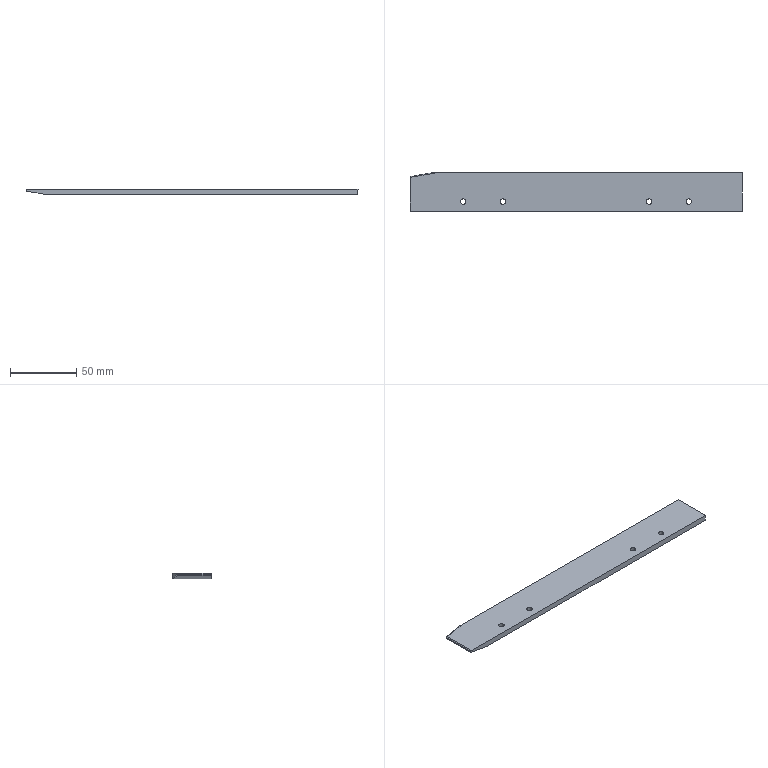Component | SolidWorks | 2SZT-0-009-3 | 1 solid | 26 faces | box 250 x 29 x 4.51 mm | volume 31578 mm3 | cylinder 15 | plane 8 | sphere 2 | spline 1 | commonest cylinder face diameters 1 x6 4.01 x4 4.2 x4 20 x1
STEP:
#1=COLOUR_RGB('',0.7922,0.8196,0.9333);
#2=FILL_AREA_STYLE_COLOUR('',#1);
#3=FILL_AREA_STYLE('',(#2));
#4=SURFACE_STYLE_FILL_AREA(#3);
#5=SURFACE_SIDE_STYLE('',(#4));
#6=SURFACE_STYLE_USAGE(.BOTH.,#5);
#7=PRESENTATION_STYLE_ASSIGNMENT((#6));
#8=CARTESIAN_POINT('',(34.695,16.445,-10.866));
#9=VERTEX_POINT('',#8);
#10=CARTESIAN_POINT('',(34.853,16.445,-10.866));
#11=VERTEX_POINT('',#10);
#12=CARTESIAN_POINT('',(34.774,16.445,-10.866));
#13=DIRECTION('',(0.00002551,0.,1.));
#14=DIRECTION('',(1.,0.,-0.00002551));
#15=AXIS2_PLACEMENT_3D('',#12,#13,#14);
#16=CIRCLE('',#15,0.07894);
#17=EDGE_CURVE('',#9,#11,#16,.T.);
#18=ORIENTED_EDGE('',*,*,#17,.F.);
#19=CARTESIAN_POINT('',(34.695,16.445,-10.689));
#20=VERTEX_POINT('',#19);
#21=CARTESIAN_POINT('',(34.695,16.445,-10.689));
#22=DIRECTION('',(0.00002551,0.,1.));
#23=VECTOR('',#22,39.37);
#24=LINE('',#21,#23);
#25=EDGE_CURVE('',#9,#20,#24,.T.);
#26=ORIENTED_EDGE('',*,*,#25,.T.);
#27=CARTESIAN_POINT('',(34.853,16.445,-10.689));
#28=VERTEX_POINT('',#27);
#29=CARTESIAN_POINT('',(34.774,16.445,-10.689));
#30=DIRECTION('',(0.00002551,0.,1.));
#31=DIRECTION('',(1.,0.,-0.00002551));
#32=AXIS2_PLACEMENT_3D('',#29,#30,#31);
#33=CIRCLE('',#32,0.07894);
#34=EDGE_CURVE('',#20,#28,#33,.T.);
#35=ORIENTED_EDGE('',*,*,#34,.T.);
#36=CARTESIAN_POINT('',(34.853,16.445,-10.689));
#37=DIRECTION('',(0.00002551,0.,1.));
#38=VECTOR('',#37,39.37);
#39=LINE('',#36,#38);
#40=EDGE_CURVE('',#11,#28,#39,.T.);
#41=ORIENTED_EDGE('',*,*,#40,.F.);
#42=EDGE_LOOP('',(#18,#26,#35,#41));
#43=FACE_OUTER_BOUND('',#42,.T.);
#44=CARTESIAN_POINT('',(34.774,16.445,-10.689));
#45=DIRECTION('',(0.00002551,0.,1.));
#46=DIRECTION('',(1.,0.,-0.00002551));
#47=AXIS2_PLACEMENT_3D('',#44,#45,#46);
#48=CYLINDRICAL_SURFACE('',#47,0.07894);
#49=ADVANCED_FACE('',(#43),#48,.F.);
#50=CARTESIAN_POINT('',(41.388,16.445,-10.866));
#51=VERTEX_POINT('',#50);
#52=CARTESIAN_POINT('',(41.546,16.445,-10.866));
#53=VERTEX_POINT('',#52);
#54=CARTESIAN_POINT('',(41.467,16.445,-10.866));
#55=DIRECTION('',(0.00002551,0.,1.));
#56=DIRECTION('',(1.,0.,-0.00002551));
#57=AXIS2_PLACEMENT_3D('',#54,#55,#56);
#58=CIRCLE('',#57,0.07894);
#59=EDGE_CURVE('',#51,#53,#58,.T.);
#60=ORIENTED_EDGE('',*,*,#59,.F.);
#61=CARTESIAN_POINT('',(41.388,16.445,-10.689));
#62=VERTEX_POINT('',#61);
#63=CARTESIAN_POINT('',(41.388,16.445,-10.689));
#64=DIRECTION('',(0.00002551,0.,1.));
#65=VECTOR('',#64,39.37);
#66=LINE('',#63,#65);
#67=EDGE_CURVE('',#51,#62,#66,.T.);
#68=ORIENTED_EDGE('',*,*,#67,.T.);
#69=CARTESIAN_POINT('',(41.546,16.445,-10.689));
#70=VERTEX_POINT('',#69);
#71=CARTESIAN_POINT('',(41.467,16.445,-10.689));
#72=DIRECTION('',(0.00002551,0.,1.));
#73=DIRECTION('',(1.,0.,-0.00002551));
#74=AXIS2_PLACEMENT_3D('',#71,#72,#73);
#75=CIRCLE('',#74,0.07894);
#76=EDGE_CURVE('',#62,#70,#75,.T.);
#77=ORIENTED_EDGE('',*,*,#76,.T.);
#78=CARTESIAN_POINT('',(41.546,16.445,-10.689));
#79=DIRECTION('',(0.00002551,0.,1.));
#80=VECTOR('',#79,39.37);
#81=LINE('',#78,#80);
#82=EDGE_CURVE('',#53,#70,#81,.T.);
#83=ORIENTED_EDGE('',*,*,#82,.F.);
#84=EDGE_LOOP('',(#60,#68,#77,#83));
#85=FACE_OUTER_BOUND('',#84,.T.);
#86=CARTESIAN_POINT('',(41.467,16.445,-10.689));
#87=DIRECTION('',(0.00002551,0.,1.));
#88=DIRECTION('',(1.,0.,-0.00002551));
#89=AXIS2_PLACEMENT_3D('',#86,#87,#88);
#90=CYLINDRICAL_SURFACE('',#89,0.07894);
#91=ADVANCED_FACE('',(#85),#90,.F.);
#92=CARTESIAN_POINT('',(35.873,16.445,-10.689));
#93=VERTEX_POINT('',#92);
#94=CARTESIAN_POINT('',(36.038,16.445,-10.689));
#95=VERTEX_POINT('',#94);
#96=CARTESIAN_POINT('',(35.955,16.445,-10.689));
#97=DIRECTION('',(0.00002551,0.,1.));
#98=DIRECTION('',(1.,0.,-0.00002551));
#99=AXIS2_PLACEMENT_3D('',#96,#97,#98);
#100=CIRCLE('',#99,0.08268);
#101=EDGE_CURVE('',#93,#95,#100,.T.);
#102=ORIENTED_EDGE('',*,*,#101,.T.);
#103=CARTESIAN_POINT('',(36.038,16.445,-10.866));
#104=VERTEX_POINT('',#103);
#105=CARTESIAN_POINT('',(36.038,16.445,-10.866));
#106=DIRECTION('',(-0.00002551,-0.,-1.));
#107=VECTOR('',#106,39.37);
#108=LINE('',#105,#107);
#109=EDGE_CURVE('',#95,#104,#108,.T.);
#110=ORIENTED_EDGE('',*,*,#109,.T.);
#111=CARTESIAN_POINT('',(35.873,16.445,-10.866));
#112=VERTEX_POINT('',#111);
#113=CARTESIAN_POINT('',(35.955,16.445,-10.866));
#114=DIRECTION('',(-0.00002551,-0.,-1.));
#115=DIRECTION('',(-1.,0.,0.00002551));
#116=AXIS2_PLACEMENT_3D('',#113,#114,#115);
#117=CIRCLE('',#116,0.08268);
#118=EDGE_CURVE('',#104,#112,#117,.T.);
#119=ORIENTED_EDGE('',*,*,#118,.T.);
#120=CARTESIAN_POINT('',(35.873,16.445,-10.866));
#121=DIRECTION('',(-0.00002551,-0.,-1.));
#122=VECTOR('',#121,39.37);
#123=LINE('',#120,#122);
#124=EDGE_CURVE('',#93,#112,#123,.T.);
#125=ORIENTED_EDGE('',*,*,#124,.F.);
#126=EDGE_LOOP('',(#102,#110,#119,#125));
#127=FACE_OUTER_BOUND('',#126,.T.);
#128=CARTESIAN_POINT('',(35.955,16.445,-10.866));
#129=DIRECTION('',(-0.00002551,-0.,-1.));
#130=DIRECTION('',(-1.,0.,0.00002551));
#131=AXIS2_PLACEMENT_3D('',#128,#129,#130);
#132=CYLINDRICAL_SURFACE('',#131,0.08268);
#133=ADVANCED_FACE('',(#127),#132,.F.);
#134=CARTESIAN_POINT('',(40.203,16.445,-10.689));
#135=VERTEX_POINT('',#134);
#136=CARTESIAN_POINT('',(40.369,16.445,-10.689));
#137=VERTEX_POINT('',#136);
#138=CARTESIAN_POINT('',(40.286,16.445,-10.689));
#139=DIRECTION('',(0.00002551,0.,1.));
#140=DIRECTION('',(1.,0.,-0.00002551));
#141=AXIS2_PLACEMENT_3D('',#138,#139,#140);
#142=CIRCLE('',#141,0.08268);
#143=EDGE_CURVE('',#135,#137,#142,.T.);
#144=ORIENTED_EDGE('',*,*,#143,.T.);
#145=CARTESIAN_POINT('',(40.369,16.445,-10.866));
#146=VERTEX_POINT('',#145);
#147=CARTESIAN_POINT('',(40.369,16.445,-10.866));
#148=DIRECTION('',(-0.00002551,-0.,-1.));
#149=VECTOR('',#148,39.37);
#150=LINE('',#147,#149);
#151=EDGE_CURVE('',#137,#146,#150,.T.);
#152=ORIENTED_EDGE('',*,*,#151,.T.);
#153=CARTESIAN_POINT('',(40.203,16.445,-10.866));
#154=VERTEX_POINT('',#153);
#155=CARTESIAN_POINT('',(40.286,16.445,-10.866));
#156=DIRECTION('',(-0.00002551,-0.,-1.));
#157=DIRECTION('',(-1.,0.,0.00002551));
#158=AXIS2_PLACEMENT_3D('',#155,#156,#157);
#159=CIRCLE('',#158,0.08268);
#160=EDGE_CURVE('',#146,#154,#159,.T.);
#161=ORIENTED_EDGE('',*,*,#160,.T.);
#162=CARTESIAN_POINT('',(40.203,16.445,-10.866));
#163=DIRECTION('',(-0.00002551,-0.,-1.));
#164=VECTOR('',#163,39.37);
#165=LINE('',#162,#164);
#166=EDGE_CURVE('',#135,#154,#165,.T.);
#167=ORIENTED_EDGE('',*,*,#166,.F.);
#168=EDGE_LOOP('',(#144,#152,#161,#167));
#169=FACE_OUTER_BOUND('',#168,.T.);
#170=CARTESIAN_POINT('',(40.286,16.445,-10.866));
#171=DIRECTION('',(-0.00002551,-0.,-1.));
#172=DIRECTION('',(-1.,0.,0.00002551));
#173=AXIS2_PLACEMENT_3D('',#170,#171,#172);
#174=CYLINDRICAL_SURFACE('',#173,0.08268);
#175=ADVANCED_FACE('',(#169),#174,.F.);
#176=CARTESIAN_POINT('',(43.042,17.302,-10.689));
#177=VERTEX_POINT('',#176);
#178=CARTESIAN_POINT('',(43.042,16.16,-10.689));
#179=VERTEX_POINT('',#178);
#180=CARTESIAN_POINT('',(43.042,16.16,-10.689));
#181=DIRECTION('',(-0.,-1.,0.));
#182=VECTOR('',#181,39.37);
#183=LINE('',#180,#182);
#184=EDGE_CURVE('',#177,#179,#183,.T.);
#185=ORIENTED_EDGE('',*,*,#184,.T.);
#186=CARTESIAN_POINT('',(43.042,16.16,-10.866));
#187=VERTEX_POINT('',#186);
#188=CARTESIAN_POINT('',(43.042,16.16,-10.866));
#189=DIRECTION('',(0.00002551,0.,1.));
#190=VECTOR('',#189,39.37);
#191=LINE('',#188,#190);
#192=EDGE_CURVE('',#187,#179,#191,.T.);
#193=ORIENTED_EDGE('',*,*,#192,.F.);
#194=CARTESIAN_POINT('',(43.042,17.302,-10.866));
#195=VERTEX_POINT('',#194);
#196=CARTESIAN_POINT('',(43.042,16.16,-10.866));
#197=DIRECTION('',(-0.,-1.,0.));
#198=VECTOR('',#197,39.37);
#199=LINE('',#196,#198);
#200=EDGE_CURVE('',#195,#187,#199,.T.);
#201=ORIENTED_EDGE('',*,*,#200,.F.);
#202=CARTESIAN_POINT('',(43.042,17.302,-10.866));
#203=DIRECTION('',(0.00002551,0.,1.));
#204=VECTOR('',#203,39.37);
#205=LINE('',#202,#204);
#206=EDGE_CURVE('',#195,#177,#205,.T.);
#207=ORIENTED_EDGE('',*,*,#206,.T.);
#208=EDGE_LOOP('',(#185,#193,#201,#207));
#209=FACE_OUTER_BOUND('',#208,.T.);
#210=CARTESIAN_POINT('',(43.042,16.16,-10.866));
#211=DIRECTION('',(-1.,0.,0.00002551));
#212=DIRECTION('',(0.00002551,0.,1.));
#213=AXIS2_PLACEMENT_3D('',#210,#211,#212);
#214=PLANE('',#213);
#215=ADVANCED_FACE('',(#209),#214,.F.);
#216=CARTESIAN_POINT('',(33.219,16.16,-10.689));
#217=VERTEX_POINT('',#216);
#218=CARTESIAN_POINT('',(43.042,16.16,-10.689));
#219=DIRECTION('',(-1.,0.,0.00002551));
#220=VECTOR('',#219,39.37);
#221=LINE('',#218,#220);
#222=EDGE_CURVE('',#179,#217,#221,.T.);
#223=ORIENTED_EDGE('',*,*,#222,.T.);
#224=CARTESIAN_POINT('',(33.199,16.16,-10.708));
#225=VERTEX_POINT('',#224);
#226=CARTESIAN_POINT('',(33.219,16.16,-10.708));
#227=DIRECTION('',(-0.,-1.,0.));
#228=DIRECTION('',(-0.00002551,0.,-1.));
#229=AXIS2_PLACEMENT_3D('',#226,#227,#228);
#230=CIRCLE('',#229,0.01969);
#231=EDGE_CURVE('',#217,#225,#230,.T.);
#232=ORIENTED_EDGE('',*,*,#231,.T.);
#233=CARTESIAN_POINT('',(33.199,16.16,-10.731));
#234=VERTEX_POINT('',#233);
#235=CARTESIAN_POINT('',(33.199,16.16,-10.866));
#236=DIRECTION('',(0.00002551,0.,1.));
#237=VECTOR('',#236,39.37);
#238=LINE('',#235,#237);
#239=EDGE_CURVE('',#234,#225,#238,.T.);
#240=ORIENTED_EDGE('',*,*,#239,.F.);
#241=CARTESIAN_POINT('',(33.216,16.16,-10.751));
#242=VERTEX_POINT('',#241);
#243=CARTESIAN_POINT('',(33.219,16.16,-10.731));
#244=DIRECTION('',(-0.,-1.,0.));
#245=DIRECTION('',(-0.00002551,0.,-1.));
#246=AXIS2_PLACEMENT_3D('',#243,#244,#245);
#247=CIRCLE('',#246,0.01969);
#248=EDGE_CURVE('',#234,#242,#247,.T.);
#249=ORIENTED_EDGE('',*,*,#248,.T.);
#250=CARTESIAN_POINT('',(33.835,16.16,-10.86));
#251=VERTEX_POINT('',#250);
#252=CARTESIAN_POINT('',(33.869,16.16,-10.866));
#253=DIRECTION('',(0.9848,-0.,-0.1737));
#254=VECTOR('',#253,39.37);
#255=LINE('',#252,#254);
#256=EDGE_CURVE('',#242,#251,#255,.T.);
#257=ORIENTED_EDGE('',*,*,#256,.T.);
#258=CARTESIAN_POINT('',(33.904,16.16,-10.866));
#259=VERTEX_POINT('',#258);
#260=CARTESIAN_POINT('',(33.904,16.16,-10.472));
#261=DIRECTION('',(-0.,-1.,0.));
#262=DIRECTION('',(-0.00002551,0.,-1.));
#263=AXIS2_PLACEMENT_3D('',#260,#261,#262);
#264=CIRCLE('',#263,0.3937);
#265=EDGE_CURVE('',#251,#259,#264,.T.);
#266=ORIENTED_EDGE('',*,*,#265,.T.);
#267=CARTESIAN_POINT('',(43.042,16.16,-10.866));
#268=DIRECTION('',(-1.,0.,0.00002551));
#269=VECTOR('',#268,39.37);
#270=LINE('',#267,#269);
#271=EDGE_CURVE('',#187,#259,#270,.T.);
#272=ORIENTED_EDGE('',*,*,#271,.F.);
#273=ORIENTED_EDGE('',*,*,#192,.T.);
#274=EDGE_LOOP('',(#223,#232,#240,#249,#257,#266,#272,#273));
#275=FACE_OUTER_BOUND('',#274,.T.);
#276=CARTESIAN_POINT('',(43.042,16.16,-10.866));
#277=DIRECTION('',(0.,1.,-0.));
#278=DIRECTION('',(-0.00002551,-0.,-1.));
#279=AXIS2_PLACEMENT_3D('',#276,#277,#278);
#280=PLANE('',#279);
#281=ADVANCED_FACE('',(#275),#280,.F.);
#282=CARTESIAN_POINT('',(33.199,17.167,-10.708));
#283=VERTEX_POINT('',#282);
#284=CARTESIAN_POINT('',(33.199,17.184,-10.708));
#285=DIRECTION('',(0.,1.,-0.));
#286=VECTOR('',#285,39.37);
#287=LINE('',#284,#286);
#288=EDGE_CURVE('',#225,#283,#287,.T.);
#289=ORIENTED_EDGE('',*,*,#288,.T.);
#290=CARTESIAN_POINT('',(33.199,17.167,-10.731));
#291=VERTEX_POINT('',#290);
#292=CARTESIAN_POINT('',(33.199,17.167,-10.731));
#293=DIRECTION('',(-0.00002551,-0.,-1.));
#294=VECTOR('',#293,39.37);
#295=LINE('',#292,#294);
#296=EDGE_CURVE('',#283,#291,#295,.T.);
#297=ORIENTED_EDGE('',*,*,#296,.T.);
#298=CARTESIAN_POINT('',(33.199,16.16,-10.731));
#299=DIRECTION('',(-0.,-1.,0.));
#300=VECTOR('',#299,39.37);
#301=LINE('',#298,#300);
#302=EDGE_CURVE('',#291,#234,#301,.T.);
#303=ORIENTED_EDGE('',*,*,#302,.T.);
#304=ORIENTED_EDGE('',*,*,#239,.T.);
#305=EDGE_LOOP('',(#289,#297,#303,#304));
#306=FACE_OUTER_BOUND('',#305,.T.);
#307=CARTESIAN_POINT('',(33.199,16.16,-10.866));
#308=DIRECTION('',(1.,-0.,-0.00002551));
#309=DIRECTION('',(-0.00002551,-0.,-1.));
#310=AXIS2_PLACEMENT_3D('',#307,#308,#309);
#311=PLANE('',#310);
#312=ADVANCED_FACE('',(#306),#311,.F.);
#313=CARTESIAN_POINT('',(33.983,17.302,-10.866));
#314=VERTEX_POINT('',#313);
#315=CARTESIAN_POINT('',(33.901,17.302,-10.86));
#316=VERTEX_POINT('',#315);
#317=CARTESIAN_POINT('',(33.983,17.302,-10.866));
#318=CARTESIAN_POINT('',(33.952,17.302,-10.866));
#319=CARTESIAN_POINT('',(33.923,17.302,-10.864));
#320=CARTESIAN_POINT('',(33.901,17.302,-10.86));
#321=(BOUNDED_CURVE()B_SPLINE_CURVE(3,(#317,#318,#319,#320),.UNSPECIFIED.,.F.,.T.)B_SPLINE_CURVE_WITH_KNOTS((4,4),(4.712,5.513),.UNSPECIFIED.)CURVE()GEOMETRIC_REPRESENTATION_ITEM()RATIONAL_B_SPLINE_CURVE((1.,0.9473,0.9473,1.))REPRESENTATION_ITEM(''));
#322=EDGE_CURVE('',#314,#316,#321,.T.);
#323=ORIENTED_EDGE('',*,*,#322,.T.);
#324=CARTESIAN_POINT('',(33.869,17.302,-10.845));
#325=VERTEX_POINT('',#324);
#326=CARTESIAN_POINT('',(33.901,17.302,-10.86));
#327=CARTESIAN_POINT('',(33.895,17.302,-10.859));
#328=CARTESIAN_POINT('',(33.889,17.302,-10.857));
#329=CARTESIAN_POINT('',(33.881,17.302,-10.854));
#330=CARTESIAN_POINT('',(33.878,17.302,-10.853));
#331=CARTESIAN_POINT('',(33.874,17.302,-10.851));
#332=CARTESIAN_POINT('',(33.873,17.302,-10.85));
#333=CARTESIAN_POINT('',(33.87,17.302,-10.848));
#334=CARTESIAN_POINT('',(33.869,17.302,-10.846));
#335=CARTESIAN_POINT('',(33.869,17.302,-10.845));
#336=B_SPLINE_CURVE_WITH_KNOTS('',3,(#326,#327,#328,#329,#330,#331,#332,#333,#334,#335),.UNSPECIFIED.,.F.,.F.,(4,2,2,2,4),(0.,0.000467,0.0007005,0.0008173,0.0009341),.UNSPECIFIED.);
#337=EDGE_CURVE('',#316,#325,#336,.T.);
#338=ORIENTED_EDGE('',*,*,#337,.T.);
#339=CARTESIAN_POINT('',(33.869,17.302,-10.708));
#340=VERTEX_POINT('',#339);
#341=CARTESIAN_POINT('',(33.869,17.302,-10.866));
#342=DIRECTION('',(0.00002551,0.,1.));
#343=VECTOR('',#342,39.37);
#344=LINE('',#341,#343);
#345=EDGE_CURVE('',#325,#340,#344,.T.);
#346=ORIENTED_EDGE('',*,*,#345,.T.);
#347=CARTESIAN_POINT('',(33.983,17.302,-10.689));
#348=VERTEX_POINT('',#347);
#349=CARTESIAN_POINT('',(33.869,17.302,-10.708));
#350=CARTESIAN_POINT('',(33.869,17.302,-10.697));
#351=CARTESIAN_POINT('',(33.916,17.302,-10.689));
#352=CARTESIAN_POINT('',(33.983,17.302,-10.689));
#353=(BOUNDED_CURVE()B_SPLINE_CURVE(3,(#349,#350,#351,#352),.UNSPECIFIED.,.F.,.T.)B_SPLINE_CURVE_WITH_KNOTS((4,4),(3.142,4.712),.UNSPECIFIED.)CURVE()GEOMETRIC_REPRESENTATION_ITEM()RATIONAL_B_SPLINE_CURVE((1.,0.8047,0.8047,1.))REPRESENTATION_ITEM(''));
#354=EDGE_CURVE('',#340,#348,#353,.T.);
#355=ORIENTED_EDGE('',*,*,#354,.T.);
#356=CARTESIAN_POINT('',(43.042,17.302,-10.689));
#357=DIRECTION('',(1.,-0.,-0.00002551));
#358=VECTOR('',#357,39.37);
#359=LINE('',#356,#358);
#360=EDGE_CURVE('',#348,#177,#359,.T.);
#361=ORIENTED_EDGE('',*,*,#360,.T.);
#362=ORIENTED_EDGE('',*,*,#206,.F.);
#363=CARTESIAN_POINT('',(43.042,17.302,-10.866));
#364=DIRECTION('',(1.,-0.,-0.00002551));
#365=VECTOR('',#364,39.37);
#366=LINE('',#363,#365);
#367=EDGE_CURVE('',#314,#195,#366,.T.);
#368=ORIENTED_EDGE('',*,*,#367,.F.);
#369=EDGE_LOOP('',(#323,#338,#346,#355,#361,#362,#368));
#370=FACE_OUTER_BOUND('',#369,.T.);
#371=CARTESIAN_POINT('',(43.042,17.302,-10.866));
#372=DIRECTION('',(-0.,-1.,0.));
#373=DIRECTION('',(0.00002551,0.,1.));
#374=AXIS2_PLACEMENT_3D('',#371,#372,#373);
#375=PLANE('',#374);
#376=ADVANCED_FACE('',(#370),#375,.F.);
#377=CARTESIAN_POINT('',(34.774,16.445,-10.866));
#378=DIRECTION('',(0.00002551,0.,1.));
#379=DIRECTION('',(1.,0.,-0.00002551));
#380=AXIS2_PLACEMENT_3D('',#377,#378,#379);
#381=CIRCLE('',#380,0.07894);
#382=EDGE_CURVE('',#11,#9,#381,.T.);
#383=ORIENTED_EDGE('',*,*,#382,.T.);
#384=ORIENTED_EDGE('',*,*,#17,.T.);
#385=EDGE_LOOP('',(#383,#384));
#386=FACE_BOUND('',#385,.T.);
#387=CARTESIAN_POINT('',(41.467,16.445,-10.866));
#388=DIRECTION('',(0.00002551,0.,1.));
#389=DIRECTION('',(1.,0.,-0.00002551));
#390=AXIS2_PLACEMENT_3D('',#387,#388,#389);
#391=CIRCLE('',#390,0.07894);
#392=EDGE_CURVE('',#53,#51,#391,.T.);
#393=ORIENTED_EDGE('',*,*,#392,.T.);
#394=ORIENTED_EDGE('',*,*,#59,.T.);
#395=EDGE_LOOP('',(#393,#394));
#396=FACE_BOUND('',#395,.T.);
#397=CARTESIAN_POINT('',(35.955,16.445,-10.866));
#398=DIRECTION('',(-0.00002551,-0.,-1.));
#399=DIRECTION('',(-1.,0.,0.00002551));
#400=AXIS2_PLACEMENT_3D('',#397,#398,#399);
#401=CIRCLE('',#400,0.08268);
#402=EDGE_CURVE('',#112,#104,#401,.T.);
#403=ORIENTED_EDGE('',*,*,#402,.F.);
#404=ORIENTED_EDGE('',*,*,#118,.F.);
#405=EDGE_LOOP('',(#403,#404));
#406=FACE_BOUND('',#405,.T.);
#407=CARTESIAN_POINT('',(40.286,16.445,-10.866));
#408=DIRECTION('',(-0.00002551,-0.,-1.));
#409=DIRECTION('',(-1.,0.,0.00002551));
#410=AXIS2_PLACEMENT_3D('',#407,#408,#409);
#411=CIRCLE('',#410,0.08268);
#412=EDGE_CURVE('',#154,#146,#411,.T.);
#413=ORIENTED_EDGE('',*,*,#412,.F.);
#414=ORIENTED_EDGE('',*,*,#160,.F.);
#415=EDGE_LOOP('',(#413,#414));
#416=FACE_BOUND('',#415,.T.);
#417=CARTESIAN_POINT('',(33.904,17.288,-10.866));
#418=VERTEX_POINT('',#417);
#419=CARTESIAN_POINT('',(33.904,17.302,-10.866));
#420=DIRECTION('',(0.,1.,-0.));
#421=VECTOR('',#420,39.37);
#422=LINE('',#419,#421);
#423=EDGE_CURVE('',#259,#418,#422,.T.);
#424=ORIENTED_EDGE('',*,*,#423,.T.);
#425=CARTESIAN_POINT('',(33.873,17.282,-10.866));
#426=DIRECTION('',(0.9848,0.1736,-0.00002512));
#427=VECTOR('',#426,39.37);
#428=LINE('',#425,#427);
#429=EDGE_CURVE('',#418,#314,#428,.T.);
#430=ORIENTED_EDGE('',*,*,#429,.T.);
#431=ORIENTED_EDGE('',*,*,#367,.T.);
#432=ORIENTED_EDGE('',*,*,#200,.T.);
#433=ORIENTED_EDGE('',*,*,#271,.T.);
#434=EDGE_LOOP('',(#424,#430,#431,#432,#433));
#435=FACE_OUTER_BOUND('',#434,.T.);
#436=CARTESIAN_POINT('',(43.042,16.16,-10.866));
#437=DIRECTION('',(0.00002551,0.,1.));
#438=DIRECTION('',(1.,-0.,-0.00002551));
#439=AXIS2_PLACEMENT_3D('',#436,#437,#438);
#440=PLANE('',#439);
#441=ADVANCED_FACE('',(#386,#396,#406,#416,#435),#440,.F.);
#442=CARTESIAN_POINT('',(34.774,16.445,-10.689));
#443=DIRECTION('',(0.00002551,0.,1.));
#444=DIRECTION('',(1.,0.,-0.00002551));
#445=AXIS2_PLACEMENT_3D('',#442,#443,#444);
#446=CIRCLE('',#445,0.07894);
#447=EDGE_CURVE('',#28,#20,#446,.T.);
#448=ORIENTED_EDGE('',*,*,#447,.F.);
#449=ORIENTED_EDGE('',*,*,#34,.F.);
#450=EDGE_LOOP('',(#448,#449));
#451=FACE_BOUND('',#450,.T.);
#452=CARTESIAN_POINT('',(41.467,16.445,-10.689));
#453=DIRECTION('',(0.00002551,0.,1.));
#454=DIRECTION('',(1.,0.,-0.00002551));
#455=AXIS2_PLACEMENT_3D('',#452,#453,#454);
#456=CIRCLE('',#455,0.07894);
#457=EDGE_CURVE('',#70,#62,#456,.T.);
#458=ORIENTED_EDGE('',*,*,#457,.F.);
#459=ORIENTED_EDGE('',*,*,#76,.F.);
#460=EDGE_LOOP('',(#458,#459));
#461=FACE_BOUND('',#460,.T.);
#462=ORIENTED_EDGE('',*,*,#101,.F.);
#463=CARTESIAN_POINT('',(35.955,16.445,-10.689));
#464=DIRECTION('',(0.00002551,0.,1.));
#465=DIRECTION('',(1.,0.,-0.00002551));
#466=AXIS2_PLACEMENT_3D('',#463,#464,#465);
#467=CIRCLE('',#466,0.08268);
#468=EDGE_CURVE('',#95,#93,#467,.T.);
#469=ORIENTED_EDGE('',*,*,#468,.F.);
#470=EDGE_LOOP('',(#462,#469));
#471=FACE_BOUND('',#470,.T.);
#472=ORIENTED_EDGE('',*,*,#143,.F.);
#473=CARTESIAN_POINT('',(40.286,16.445,-10.689));
#474=DIRECTION('',(0.00002551,0.,1.));
#475=DIRECTION('',(1.,0.,-0.00002551));
#476=AXIS2_PLACEMENT_3D('',#473,#474,#475);
#477=CIRCLE('',#476,0.08268);
#478=EDGE_CURVE('',#137,#135,#477,.T.);
#479=ORIENTED_EDGE('',*,*,#478,.F.);
#480=EDGE_LOOP('',(#472,#479));
#481=FACE_BOUND('',#480,.T.);
#482=ORIENTED_EDGE('',*,*,#360,.F.);
#483=CARTESIAN_POINT('',(33.219,17.167,-10.689));
#484=VERTEX_POINT('',#483);
#485=CARTESIAN_POINT('',(42.574,18.817,-10.689));
#486=DIRECTION('',(-0.9848,-0.1736,0.00002512));
#487=VECTOR('',#486,39.37);
#488=LINE('',#485,#487);
#489=EDGE_CURVE('',#348,#484,#488,.T.);
#490=ORIENTED_EDGE('',*,*,#489,.T.);
#491=CARTESIAN_POINT('',(33.219,16.16,-10.689));
#492=DIRECTION('',(-0.,-1.,0.));
#493=VECTOR('',#492,39.37);
#494=LINE('',#491,#493);
#495=EDGE_CURVE('',#484,#217,#494,.T.);
#496=ORIENTED_EDGE('',*,*,#495,.T.);
#497=ORIENTED_EDGE('',*,*,#222,.F.);
#498=ORIENTED_EDGE('',*,*,#184,.F.);
#499=EDGE_LOOP('',(#482,#490,#496,#497,#498));
#500=FACE_OUTER_BOUND('',#499,.T.);
#501=CARTESIAN_POINT('',(43.042,16.16,-10.689));
#502=DIRECTION('',(0.00002551,0.,1.));
#503=DIRECTION('',(1.,-0.,-0.00002551));
#504=AXIS2_PLACEMENT_3D('',#501,#502,#503);
#505=PLANE('',#504);
#506=ADVANCED_FACE('',(#451,#461,#471,#481,#500),#505,.T.);
#507=ORIENTED_EDGE('',*,*,#151,.F.);
#508=ORIENTED_EDGE('',*,*,#478,.T.);
#509=ORIENTED_EDGE('',*,*,#166,.T.);
#510=ORIENTED_EDGE('',*,*,#412,.T.);
#511=EDGE_LOOP('',(#507,#508,#509,#510));
#512=FACE_OUTER_BOUND('',#511,.T.);
#513=CARTESIAN_POINT('',(40.286,16.445,-10.866));
#514=DIRECTION('',(-0.00002551,-0.,-1.));
#515=DIRECTION('',(-1.,0.,0.00002551));
#516=AXIS2_PLACEMENT_3D('',#513,#514,#515);
#517=CYLINDRICAL_SURFACE('',#516,0.08268);
#518=ADVANCED_FACE('',(#512),#517,.F.);
#519=ORIENTED_EDGE('',*,*,#109,.F.);
#520=ORIENTED_EDGE('',*,*,#468,.T.);
#521=ORIENTED_EDGE('',*,*,#124,.T.);
#522=ORIENTED_EDGE('',*,*,#402,.T.);
#523=EDGE_LOOP('',(#519,#520,#521,#522));
#524=FACE_OUTER_BOUND('',#523,.T.);
#525=CARTESIAN_POINT('',(35.955,16.445,-10.866));
#526=DIRECTION('',(-0.00002551,-0.,-1.));
#527=DIRECTION('',(-1.,0.,0.00002551));
#528=AXIS2_PLACEMENT_3D('',#525,#526,#527);
#529=CYLINDRICAL_SURFACE('',#528,0.08268);
#530=ADVANCED_FACE('',(#524),#529,.F.);
#531=ORIENTED_EDGE('',*,*,#67,.F.);
#532=ORIENTED_EDGE('',*,*,#392,.F.);
#533=ORIENTED_EDGE('',*,*,#82,.T.);
#534=ORIENTED_EDGE('',*,*,#457,.T.);
#535=EDGE_LOOP('',(#531,#532,#533,#534));
#536=FACE_OUTER_BOUND('',#535,.T.);
#537=CARTESIAN_POINT('',(41.467,16.445,-10.689));
#538=DIRECTION('',(0.00002551,0.,1.));
#539=DIRECTION('',(1.,0.,-0.00002551));
#540=AXIS2_PLACEMENT_3D('',#537,#538,#539);
#541=CYLINDRICAL_SURFACE('',#540,0.07894);
#542=ADVANCED_FACE('',(#536),#541,.F.);
#543=ORIENTED_EDGE('',*,*,#25,.F.);
#544=ORIENTED_EDGE('',*,*,#382,.F.);
#545=ORIENTED_EDGE('',*,*,#40,.T.);
#546=ORIENTED_EDGE('',*,*,#447,.T.);
#547=EDGE_LOOP('',(#543,#544,#545,#546));
#548=FACE_OUTER_BOUND('',#547,.T.);
#549=CARTESIAN_POINT('',(34.774,16.445,-10.689));
#550=DIRECTION('',(0.00002551,0.,1.));
#551=DIRECTION('',(1.,0.,-0.00002551));
#552=AXIS2_PLACEMENT_3D('',#549,#550,#551);
#553=CYLINDRICAL_SURFACE('',#552,0.07894);
#554=ADVANCED_FACE('',(#548),#553,.F.);
#555=CARTESIAN_POINT('',(33.216,17.167,-10.751));
#556=VERTEX_POINT('',#555);
#557=CARTESIAN_POINT('',(33.216,17.184,-10.751));
#558=DIRECTION('',(0.,1.,-0.));
#559=VECTOR('',#558,39.37);
#560=LINE('',#557,#559);
#561=EDGE_CURVE('',#242,#556,#560,.T.);
#562=ORIENTED_EDGE('',*,*,#561,.T.);
#563=CARTESIAN_POINT('',(33.835,17.276,-10.86));
#564=VERTEX_POINT('',#563);
#565=CARTESIAN_POINT('',(33.683,17.25,-10.833));
#566=DIRECTION('',(0.9703,0.1711,-0.1711));
#567=VECTOR('',#566,39.37);
#568=LINE('',#565,#567);
#569=EDGE_CURVE('',#556,#564,#568,.T.);
#570=ORIENTED_EDGE('',*,*,#569,.T.);
#571=CARTESIAN_POINT('',(33.835,16.16,-10.86));
#572=DIRECTION('',(-0.,-1.,0.));
#573=VECTOR('',#572,39.37);
#574=LINE('',#571,#573);
#575=EDGE_CURVE('',#564,#251,#574,.T.);
#576=ORIENTED_EDGE('',*,*,#575,.T.);
#577=ORIENTED_EDGE('',*,*,#256,.F.);
#578=EDGE_LOOP('',(#562,#570,#576,#577));
#579=FACE_OUTER_BOUND('',#578,.T.);
#580=CARTESIAN_POINT('',(33.869,16.16,-10.866));
#581=DIRECTION('',(0.1737,0.,0.9848));
#582=DIRECTION('',(0.,1.,-0.));
#583=AXIS2_PLACEMENT_3D('',#580,#581,#582);
#584=PLANE('',#583);
#585=ADVANCED_FACE('',(#579),#584,.F.);
#586=ORIENTED_EDGE('',*,*,#345,.F.);
#587=CARTESIAN_POINT('',(33.835,17.296,-10.841));
#588=VERTEX_POINT('',#587);
#589=CARTESIAN_POINT('',(33.869,17.302,-10.845));
#590=CARTESIAN_POINT('',(33.858,17.3,-10.844));
#591=CARTESIAN_POINT('',(33.847,17.298,-10.842));
#592=CARTESIAN_POINT('',(33.835,17.296,-10.841));
#593=(BOUNDED_CURVE()B_SPLINE_CURVE(3,(#589,#590,#591,#592),.UNSPECIFIED.,.F.,.F.)B_SPLINE_CURVE_WITH_KNOTS((4,4),(1.654,1.745),.UNSPECIFIED.)CURVE()GEOMETRIC_REPRESENTATION_ITEM()RATIONAL_B_SPLINE_CURVE((1.,0.9993,0.9993,1.))REPRESENTATION_ITEM(''));
#594=EDGE_CURVE('',#325,#588,#593,.T.);
#595=ORIENTED_EDGE('',*,*,#594,.T.);
#596=CARTESIAN_POINT('',(33.216,17.187,-10.731));
#597=VERTEX_POINT('',#596);
#598=CARTESIAN_POINT('',(33.873,17.302,-10.847));
#599=DIRECTION('',(-0.9703,-0.1711,0.1711));
#600=VECTOR('',#599,39.37);
#601=LINE('',#598,#600);
#602=EDGE_CURVE('',#588,#597,#601,.T.);
#603=ORIENTED_EDGE('',*,*,#602,.T.);
#604=CARTESIAN_POINT('',(33.216,17.187,-10.708));
#605=VERTEX_POINT('',#604);
#606=CARTESIAN_POINT('',(33.216,17.187,-10.708));
#607=DIRECTION('',(0.00002551,0.,1.));
#608=VECTOR('',#607,39.37);
#609=LINE('',#606,#608);
#610=EDGE_CURVE('',#597,#605,#609,.T.);
#611=ORIENTED_EDGE('',*,*,#610,.T.);
#612=CARTESIAN_POINT('',(33.869,17.302,-10.708));
#613=DIRECTION('',(0.9848,0.1736,-0.00002512));
#614=VECTOR('',#613,39.37);
#615=LINE('',#612,#614);
#616=EDGE_CURVE('',#605,#340,#615,.T.);
#617=ORIENTED_EDGE('',*,*,#616,.T.);
#618=EDGE_LOOP('',(#586,#595,#603,#611,#617));
#619=FACE_OUTER_BOUND('',#618,.T.);
#620=CARTESIAN_POINT('',(33.869,17.302,-10.866));
#621=DIRECTION('',(0.1736,-0.9848,-0.00000443));
#622=DIRECTION('',(0.00002551,0.,1.));
#623=AXIS2_PLACEMENT_3D('',#620,#621,#622);
#624=PLANE('',#623);
#625=ADVANCED_FACE('',(#619),#624,.F.);
#626=ORIENTED_EDGE('',*,*,#575,.F.);
#627=CARTESIAN_POINT('',(33.835,17.276,-10.86));
#628=CARTESIAN_POINT('',(33.858,17.28,-10.864));
#629=CARTESIAN_POINT('',(33.881,17.284,-10.866));
#630=CARTESIAN_POINT('',(33.904,17.288,-10.866));
#631=(BOUNDED_CURVE()B_SPLINE_CURVE(3,(#627,#628,#629,#630),.UNSPECIFIED.,.F.,.T.)B_SPLINE_CURVE_WITH_KNOTS((4,4),(4.538,4.712),.UNSPECIFIED.)CURVE()GEOMETRIC_REPRESENTATION_ITEM()RATIONAL_B_SPLINE_CURVE((1.,0.9975,0.9975,1.))REPRESENTATION_ITEM(''));
#632=EDGE_CURVE('',#564,#418,#631,.T.);
#633=ORIENTED_EDGE('',*,*,#632,.T.);
#634=ORIENTED_EDGE('',*,*,#423,.F.);
#635=ORIENTED_EDGE('',*,*,#265,.F.);
#636=EDGE_LOOP('',(#626,#633,#634,#635));
#637=FACE_OUTER_BOUND('',#636,.T.);
#638=CARTESIAN_POINT('',(33.904,16.16,-10.472));
#639=DIRECTION('',(0.,1.,-0.));
#640=DIRECTION('',(-0.00002551,0.,-1.));
#641=AXIS2_PLACEMENT_3D('',#638,#639,#640);
#642=CYLINDRICAL_SURFACE('',#641,0.3937);
#643=ADVANCED_FACE('',(#637),#642,.T.);
#644=ORIENTED_EDGE('',*,*,#495,.F.);
#645=CARTESIAN_POINT('',(33.219,17.167,-10.708));
#646=DIRECTION('',(-0.,-1.,0.));
#647=DIRECTION('',(0.00002551,0.,1.));
#648=AXIS2_PLACEMENT_3D('',#645,#646,#647);
#649=CIRCLE('',#648,0.01969);
#650=EDGE_CURVE('',#484,#283,#649,.T.);
#651=ORIENTED_EDGE('',*,*,#650,.T.);
#652=ORIENTED_EDGE('',*,*,#288,.F.);
#653=ORIENTED_EDGE('',*,*,#231,.F.);
#654=EDGE_LOOP('',(#644,#651,#652,#653));
#655=FACE_OUTER_BOUND('',#654,.T.);
#656=CARTESIAN_POINT('',(33.219,16.16,-10.708));
#657=DIRECTION('',(-0.,-1.,0.));
#658=DIRECTION('',(0.00002551,0.,1.));
#659=AXIS2_PLACEMENT_3D('',#656,#657,#658);
#660=CYLINDRICAL_SURFACE('',#659,0.01969);
#661=ADVANCED_FACE('',(#655),#660,.T.);
#662=ORIENTED_EDGE('',*,*,#302,.F.);
#663=CARTESIAN_POINT('',(33.219,17.167,-10.731));
#664=DIRECTION('',(-0.,-1.,0.));
#665=DIRECTION('',(0.00002551,0.,1.));
#666=AXIS2_PLACEMENT_3D('',#663,#664,#665);
#667=CIRCLE('',#666,0.01969);
#668=EDGE_CURVE('',#291,#556,#667,.T.);
#669=ORIENTED_EDGE('',*,*,#668,.T.);
#670=ORIENTED_EDGE('',*,*,#561,.F.);
#671=ORIENTED_EDGE('',*,*,#248,.F.);
#672=EDGE_LOOP('',(#662,#669,#670,#671));
#673=FACE_OUTER_BOUND('',#672,.T.);
#674=CARTESIAN_POINT('',(33.219,16.16,-10.731));
#675=DIRECTION('',(-0.,-1.,0.));
#676=DIRECTION('',(0.00002551,0.,1.));
#677=AXIS2_PLACEMENT_3D('',#674,#675,#676);
#678=CYLINDRICAL_SURFACE('',#677,0.01969);
#679=ADVANCED_FACE('',(#673),#678,.T.);
#680=CARTESIAN_POINT('',(33.219,17.167,-10.708));
#681=DIRECTION('',(-0.9848,-0.1736,0.00002512));
#682=DIRECTION('',(-0.1736,0.9848,0.00000443));
#683=AXIS2_PLACEMENT_3D('',#680,#681,#682);
#684=CIRCLE('',#683,0.01969);
#685=EDGE_CURVE('',#484,#605,#684,.T.);
#686=ORIENTED_EDGE('',*,*,#685,.F.);
#687=ORIENTED_EDGE('',*,*,#489,.F.);
#688=ORIENTED_EDGE('',*,*,#354,.F.);
#689=ORIENTED_EDGE('',*,*,#616,.F.);
#690=EDGE_LOOP('',(#686,#687,#688,#689));
#691=FACE_OUTER_BOUND('',#690,.T.);
#692=CARTESIAN_POINT('',(42.574,18.817,-10.709));
#693=DIRECTION('',(0.9848,0.1736,-0.00002512));
#694=DIRECTION('',(0.1736,-0.9848,-0.00000443));
#695=AXIS2_PLACEMENT_3D('',#692,#693,#694);
#696=CYLINDRICAL_SURFACE('',#695,0.01969);
#697=ADVANCED_FACE('',(#691),#696,.T.);
#698=ORIENTED_EDGE('',*,*,#650,.F.);
#699=ORIENTED_EDGE('',*,*,#685,.T.);
#700=CARTESIAN_POINT('',(33.219,17.167,-10.708));
#701=DIRECTION('',(-0.00002551,-0.,-1.));
#702=DIRECTION('',(-1.,0.,0.00002551));
#703=AXIS2_PLACEMENT_3D('',#700,#701,#702);
#704=CIRCLE('',#703,0.01969);
#705=EDGE_CURVE('',#283,#605,#704,.T.);
#706=ORIENTED_EDGE('',*,*,#705,.F.);
#707=EDGE_LOOP('',(#698,#699,#706));
#708=FACE_OUTER_BOUND('',#707,.T.);
#709=CARTESIAN_POINT('',(33.219,17.167,-10.708));
#710=DIRECTION('',(-0.,1.,-0.));
#711=DIRECTION('',(-1.,0.,0.00002551));
#712=AXIS2_PLACEMENT_3D('',#709,#710,#711);
#713=SPHERICAL_SURFACE('',#712,0.01969);
#714=ADVANCED_FACE('',(#708),#713,.T.);
#715=CARTESIAN_POINT('',(33.219,17.167,-10.731));
#716=DIRECTION('',(-0.00002551,-0.,-1.));
#717=DIRECTION('',(-1.,0.,0.00002551));
#718=AXIS2_PLACEMENT_3D('',#715,#716,#717);
#719=CIRCLE('',#718,0.01969);
#720=EDGE_CURVE('',#291,#597,#719,.T.);
#721=ORIENTED_EDGE('',*,*,#720,.F.);
#722=ORIENTED_EDGE('',*,*,#296,.F.);
#723=ORIENTED_EDGE('',*,*,#705,.T.);
#724=ORIENTED_EDGE('',*,*,#610,.F.);
#725=EDGE_LOOP('',(#721,#722,#723,#724));
#726=FACE_OUTER_BOUND('',#725,.T.);
#727=CARTESIAN_POINT('',(33.219,17.167,-10.866));
#728=DIRECTION('',(-0.00002551,-0.,-1.));
#729=DIRECTION('',(-1.,0.,0.00002551));
#730=AXIS2_PLACEMENT_3D('',#727,#728,#729);
#731=CYLINDRICAL_SURFACE('',#730,0.01969);
#732=ADVANCED_FACE('',(#726),#731,.T.);
#733=ORIENTED_EDGE('',*,*,#668,.F.);
#734=ORIENTED_EDGE('',*,*,#720,.T.);
#735=CARTESIAN_POINT('',(33.219,17.167,-10.731));
#736=DIRECTION('',(0.9703,0.1711,-0.1711));
#737=DIRECTION('',(0.1736,-0.9848,-0.00000443));
#738=AXIS2_PLACEMENT_3D('',#735,#736,#737);
#739=CIRCLE('',#738,0.01969);
#740=EDGE_CURVE('',#556,#597,#739,.T.);
#741=ORIENTED_EDGE('',*,*,#740,.F.);
#742=EDGE_LOOP('',(#733,#734,#741));
#743=FACE_OUTER_BOUND('',#742,.T.);
#744=CARTESIAN_POINT('',(33.219,17.167,-10.731));
#745=DIRECTION('',(-0.,1.,-0.));
#746=DIRECTION('',(-1.,0.,0.00002551));
#747=AXIS2_PLACEMENT_3D('',#744,#745,#746);
#748=SPHERICAL_SURFACE('',#747,0.01969);
#749=ADVANCED_FACE('',(#743),#748,.T.);
#750=ORIENTED_EDGE('',*,*,#740,.T.);
#751=ORIENTED_EDGE('',*,*,#602,.F.);
#752=CARTESIAN_POINT('',(33.839,17.276,-10.841));
#753=DIRECTION('',(0.9703,0.1711,-0.1711));
#754=DIRECTION('',(0.1736,-0.9848,-0.00000443));
#755=AXIS2_PLACEMENT_3D('',#752,#753,#754);
#756=CIRCLE('',#755,0.01969);
#757=EDGE_CURVE('',#564,#588,#756,.T.);
#758=ORIENTED_EDGE('',*,*,#757,.F.);
#759=ORIENTED_EDGE('',*,*,#569,.F.);
#760=EDGE_LOOP('',(#750,#751,#758,#759));
#761=FACE_OUTER_BOUND('',#760,.T.);
#762=CARTESIAN_POINT('',(33.876,17.283,-10.847));
#763=DIRECTION('',(-0.9703,-0.1711,0.1711));
#764=DIRECTION('',(0.1737,0.,0.9848));
#765=AXIS2_PLACEMENT_3D('',#762,#763,#764);
#766=CYLINDRICAL_SURFACE('',#765,0.01969);
#767=ADVANCED_FACE('',(#761),#766,.T.);
#768=ORIENTED_EDGE('',*,*,#594,.F.);
#769=ORIENTED_EDGE('',*,*,#337,.F.);
#770=CARTESIAN_POINT('',(33.904,17.288,-10.846));
#771=DIRECTION('',(0.9848,0.1736,-0.00002512));
#772=DIRECTION('',(0.1736,-0.9848,-0.00000443));
#773=AXIS2_PLACEMENT_3D('',#770,#771,#772);
#774=CIRCLE('',#773,0.01969);
#775=EDGE_CURVE('',#418,#316,#774,.T.);
#776=ORIENTED_EDGE('',*,*,#775,.F.);
#777=ORIENTED_EDGE('',*,*,#632,.F.);
#778=ORIENTED_EDGE('',*,*,#757,.T.);
#779=EDGE_LOOP('',(#768,#769,#776,#777,#778));
#780=FACE_OUTER_BOUND('',#779,.T.);
#781=CARTESIAN_POINT('',(33.835,17.296,-10.841));
#782=CARTESIAN_POINT('',(33.832,17.295,-10.859));
#783=CARTESIAN_POINT('',(33.835,17.276,-10.86));
#784=CARTESIAN_POINT('',(33.857,17.3,-10.844));
#785=CARTESIAN_POINT('',(33.855,17.299,-10.864));
#786=CARTESIAN_POINT('',(33.858,17.28,-10.864));
#787=CARTESIAN_POINT('',(33.879,17.303,-10.846));
#788=CARTESIAN_POINT('',(33.878,17.303,-10.866));
#789=CARTESIAN_POINT('',(33.881,17.284,-10.866));
#790=CARTESIAN_POINT('',(33.9,17.307,-10.846));
#791=CARTESIAN_POINT('',(33.9,17.307,-10.866));
#792=CARTESIAN_POINT('',(33.904,17.288,-10.866));
#793=(BOUNDED_SURFACE()B_SPLINE_SURFACE(3,2,((#781,#782,#783),(#784,#785,#786),(#787,#788,#789),(#790,#791,#792)),.UNSPECIFIED.,.F.,.F.,.F.)B_SPLINE_SURFACE_WITH_KNOTS((4,4),(3,3),(4.538,4.712),(0.,1.),.UNSPECIFIED.)GEOMETRIC_REPRESENTATION_ITEM()RATIONAL_B_SPLINE_SURFACE(((1.,0.7177,1.),(1.,0.7142,1.),(1.,0.7107,1.),(1.,0.7071,1.)))REPRESENTATION_ITEM('')SURFACE());
#794=ADVANCED_FACE('',(#780),#793,.T.);
#795=ORIENTED_EDGE('',*,*,#322,.F.);
#796=ORIENTED_EDGE('',*,*,#429,.F.);
#797=ORIENTED_EDGE('',*,*,#775,.T.);
#798=EDGE_LOOP('',(#795,#796,#797));
#799=FACE_OUTER_BOUND('',#798,.T.);
#800=CARTESIAN_POINT('',(33.873,17.282,-10.846));
#801=DIRECTION('',(-0.9848,-0.1736,0.00002512));
#802=DIRECTION('',(-0.1736,0.9848,0.00000443));
#803=AXIS2_PLACEMENT_3D('',#800,#801,#802);
#804=CYLINDRICAL_SURFACE('',#803,0.01969);
#805=ADVANCED_FACE('',(#799),#804,.T.);
#806=CLOSED_SHELL('',(#49,#91,#133,#175,#215,#281,#312,#376,#441,#506,#518,#530,#542,#554,#585,#625,#643,#661,#679,#697,#714,#732,#749,#767,#794,#805));
#807=MANIFOLD_SOLID_BREP('',#806);
#808=STYLED_ITEM('',(#7),#807);
#809=PRESENTATION_LAYER_ASSIGNMENT('','',(#808));
#810=(LENGTH_UNIT()NAMED_UNIT(*)SI_UNIT($,.METRE.));
#811=LENGTH_MEASURE_WITH_UNIT(LENGTH_MEASURE(0.0254),#810);
#812=DIMENSIONAL_EXPONENTS(1.,0.,0.,0.,0.,0.,0.);
#813=(CONVERSION_BASED_UNIT('',#811)LENGTH_UNIT()NAMED_UNIT(#812));
#814=UNCERTAINTY_MEASURE_WITH_UNIT(LENGTH_MEASURE(0.00001),#813,'','');
#815=(NAMED_UNIT(*)PLANE_ANGLE_UNIT()SI_UNIT($,.RADIAN.));
#816=(NAMED_UNIT(*)SI_UNIT($,.STERADIAN.)SOLID_ANGLE_UNIT());
#817=(GEOMETRIC_REPRESENTATION_CONTEXT(3)GLOBAL_UNCERTAINTY_ASSIGNED_CONTEXT((#814))GLOBAL_UNIT_ASSIGNED_CONTEXT((#813,#815,#816))REPRESENTATION_CONTEXT('',''));
#818=MECHANICAL_DESIGN_GEOMETRIC_PRESENTATION_REPRESENTATION('',(#808),#817);
#819=CARTESIAN_POINT('',(0.,0.,0.));
#820=DIRECTION('',(0.,0.,1.));
#821=DIRECTION('',(1.,0.,0.));
#822=AXIS2_PLACEMENT_3D('',#819,#820,#821);
#823=(LENGTH_UNIT()NAMED_UNIT(*)SI_UNIT($,.METRE.));
#824=LENGTH_MEASURE_WITH_UNIT(LENGTH_MEASURE(0.0254),#823);
#825=DIMENSIONAL_EXPONENTS(1.,0.,0.,0.,0.,0.,0.);
#826=(CONVERSION_BASED_UNIT('',#824)LENGTH_UNIT()NAMED_UNIT(#825));
#827=UNCERTAINTY_MEASURE_WITH_UNIT(LENGTH_MEASURE(0.00001),#826,'','');
#828=(NAMED_UNIT(*)PLANE_ANGLE_UNIT()SI_UNIT($,.RADIAN.));
#829=(NAMED_UNIT(*)SI_UNIT($,.STERADIAN.)SOLID_ANGLE_UNIT());
#830=(GEOMETRIC_REPRESENTATION_CONTEXT(3)GLOBAL_UNCERTAINTY_ASSIGNED_CONTEXT((#827))GLOBAL_UNIT_ASSIGNED_CONTEXT((#826,#828,#829))REPRESENTATION_CONTEXT('',''));
#831=ADVANCED_BREP_SHAPE_REPRESENTATION('',(#807,#822),#830);